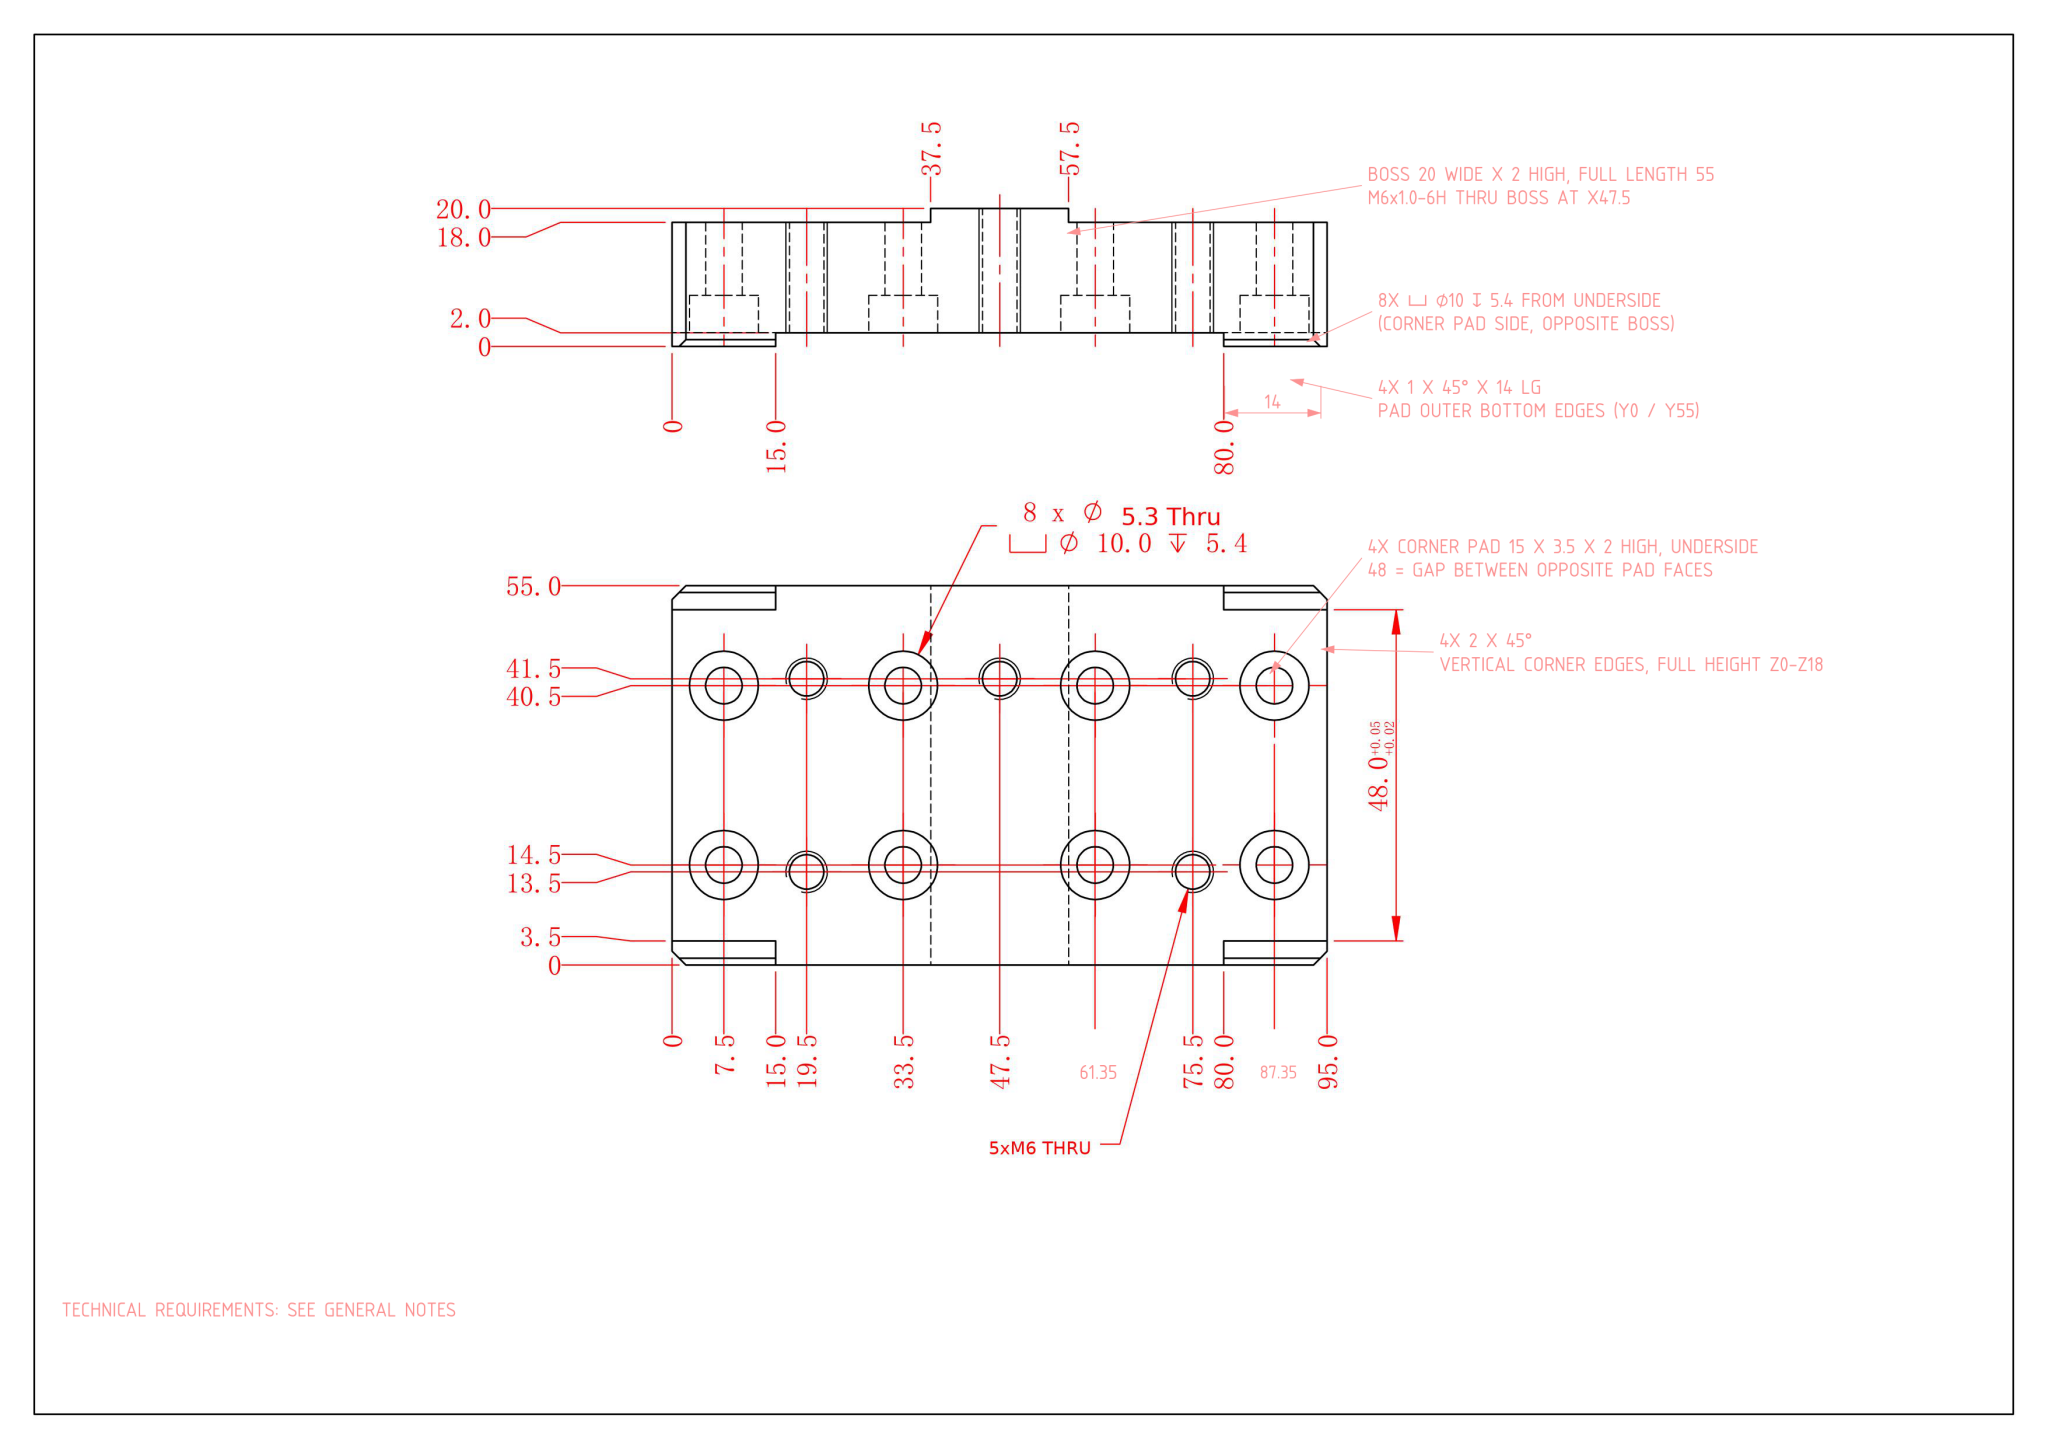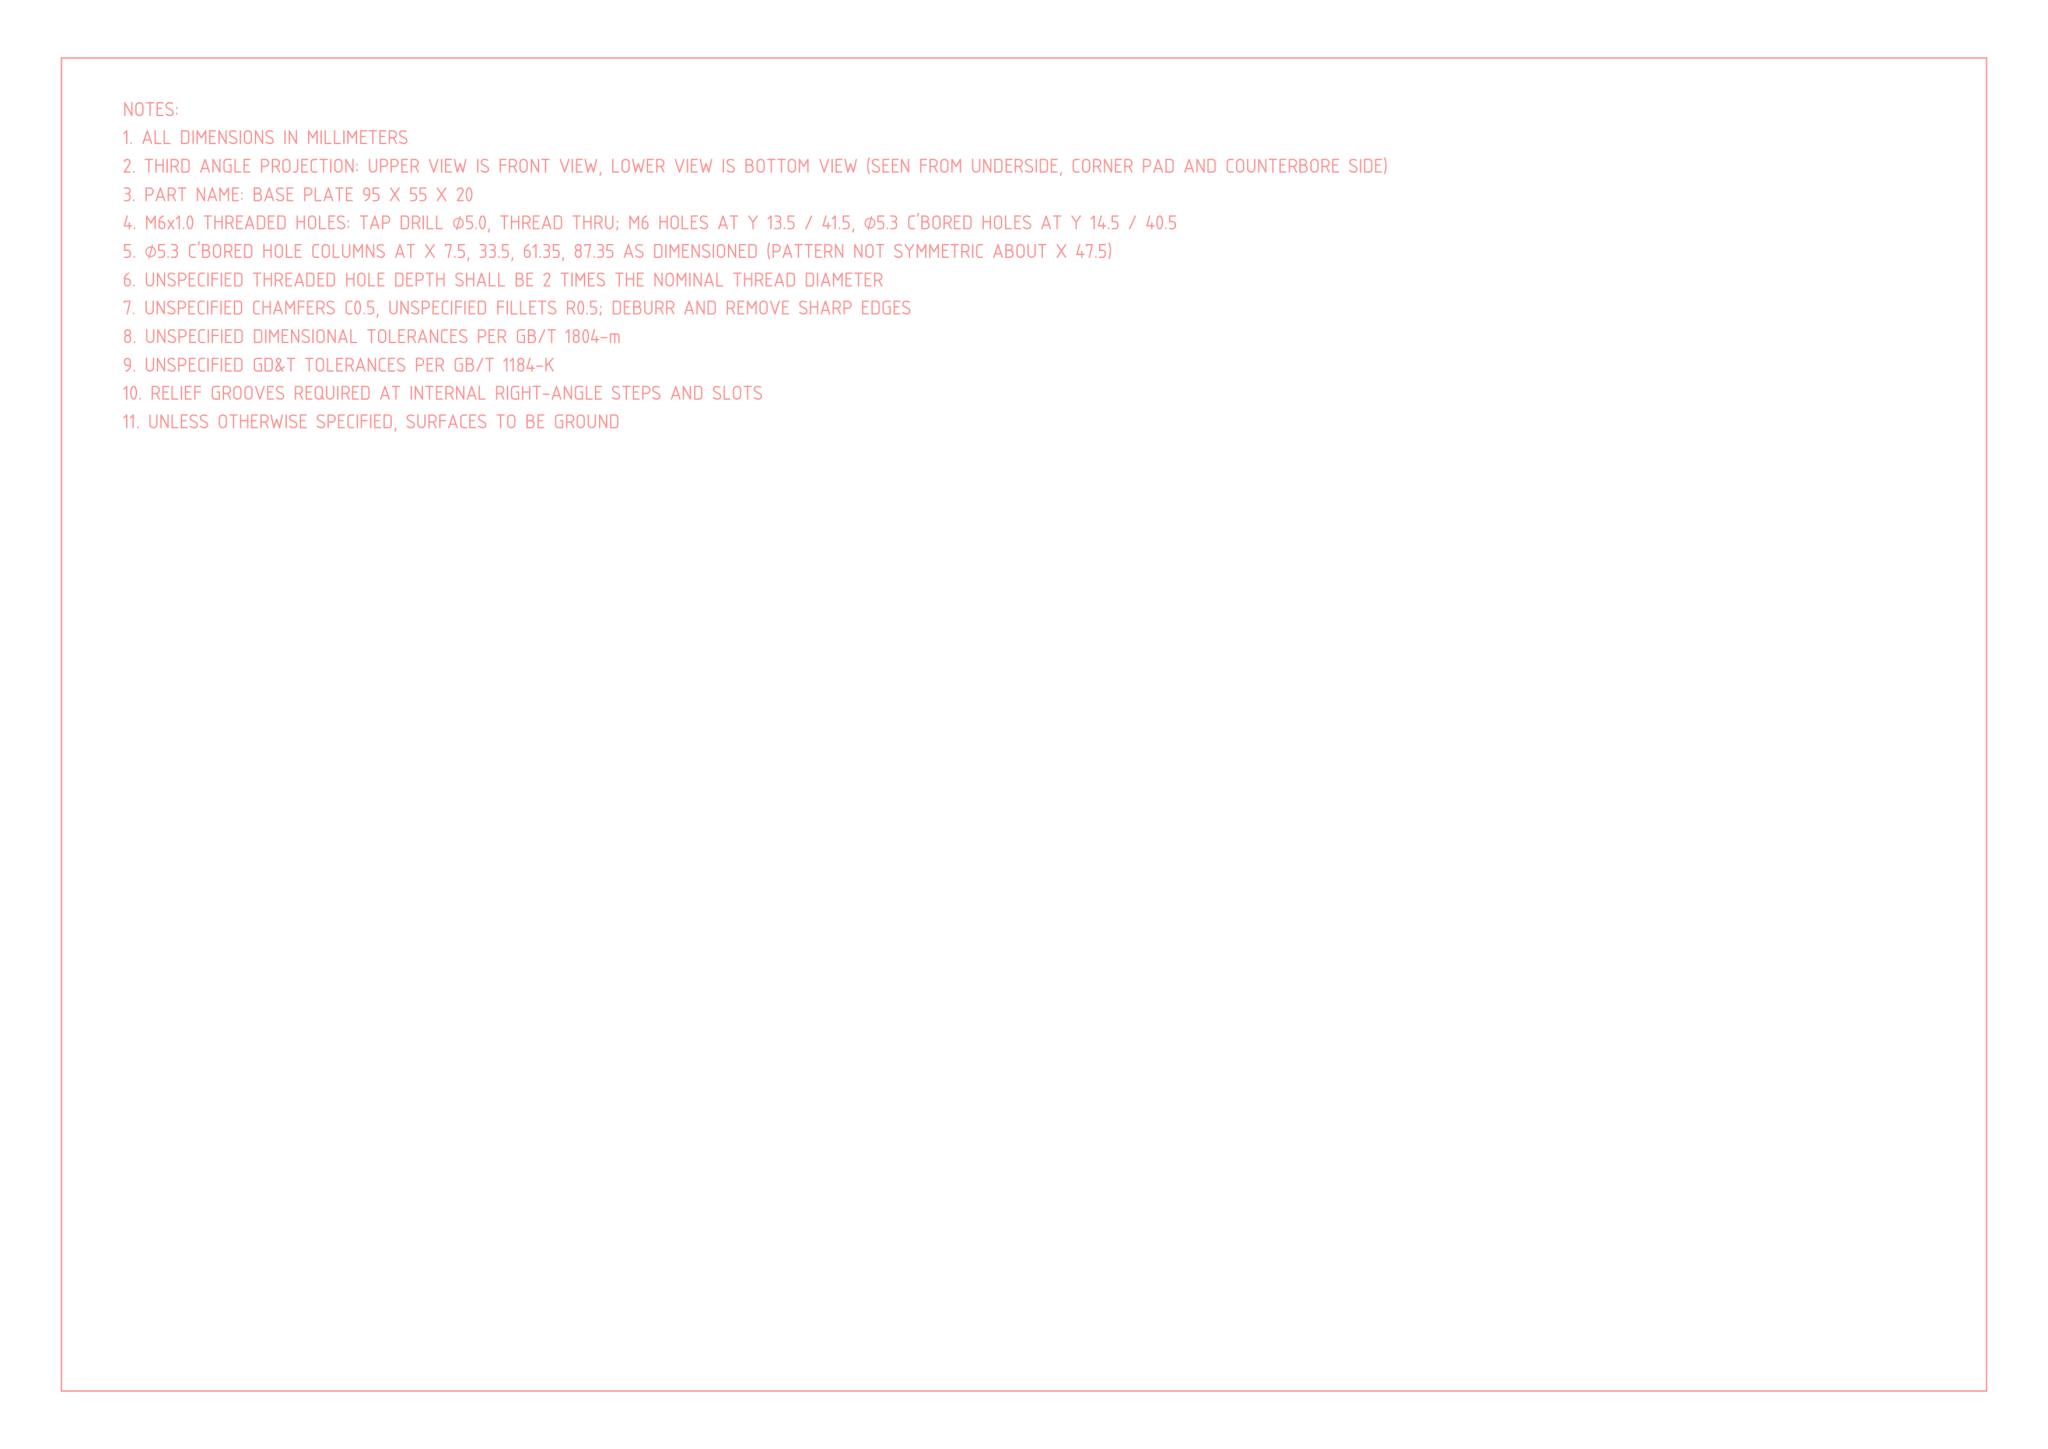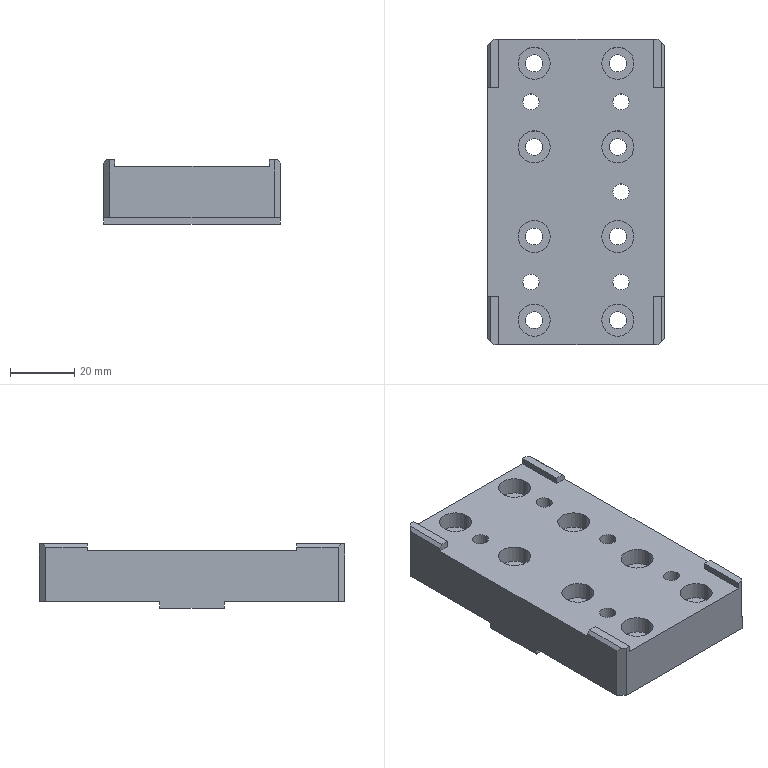Part | NX | mm | 1 solid | 80 faces | box 55 x 95 x 20 mm | volume 79176 mm3 | cylinder 42 | plane 38 | commonest cylinder face diameters 10 x16 5.3 x16 5 x10